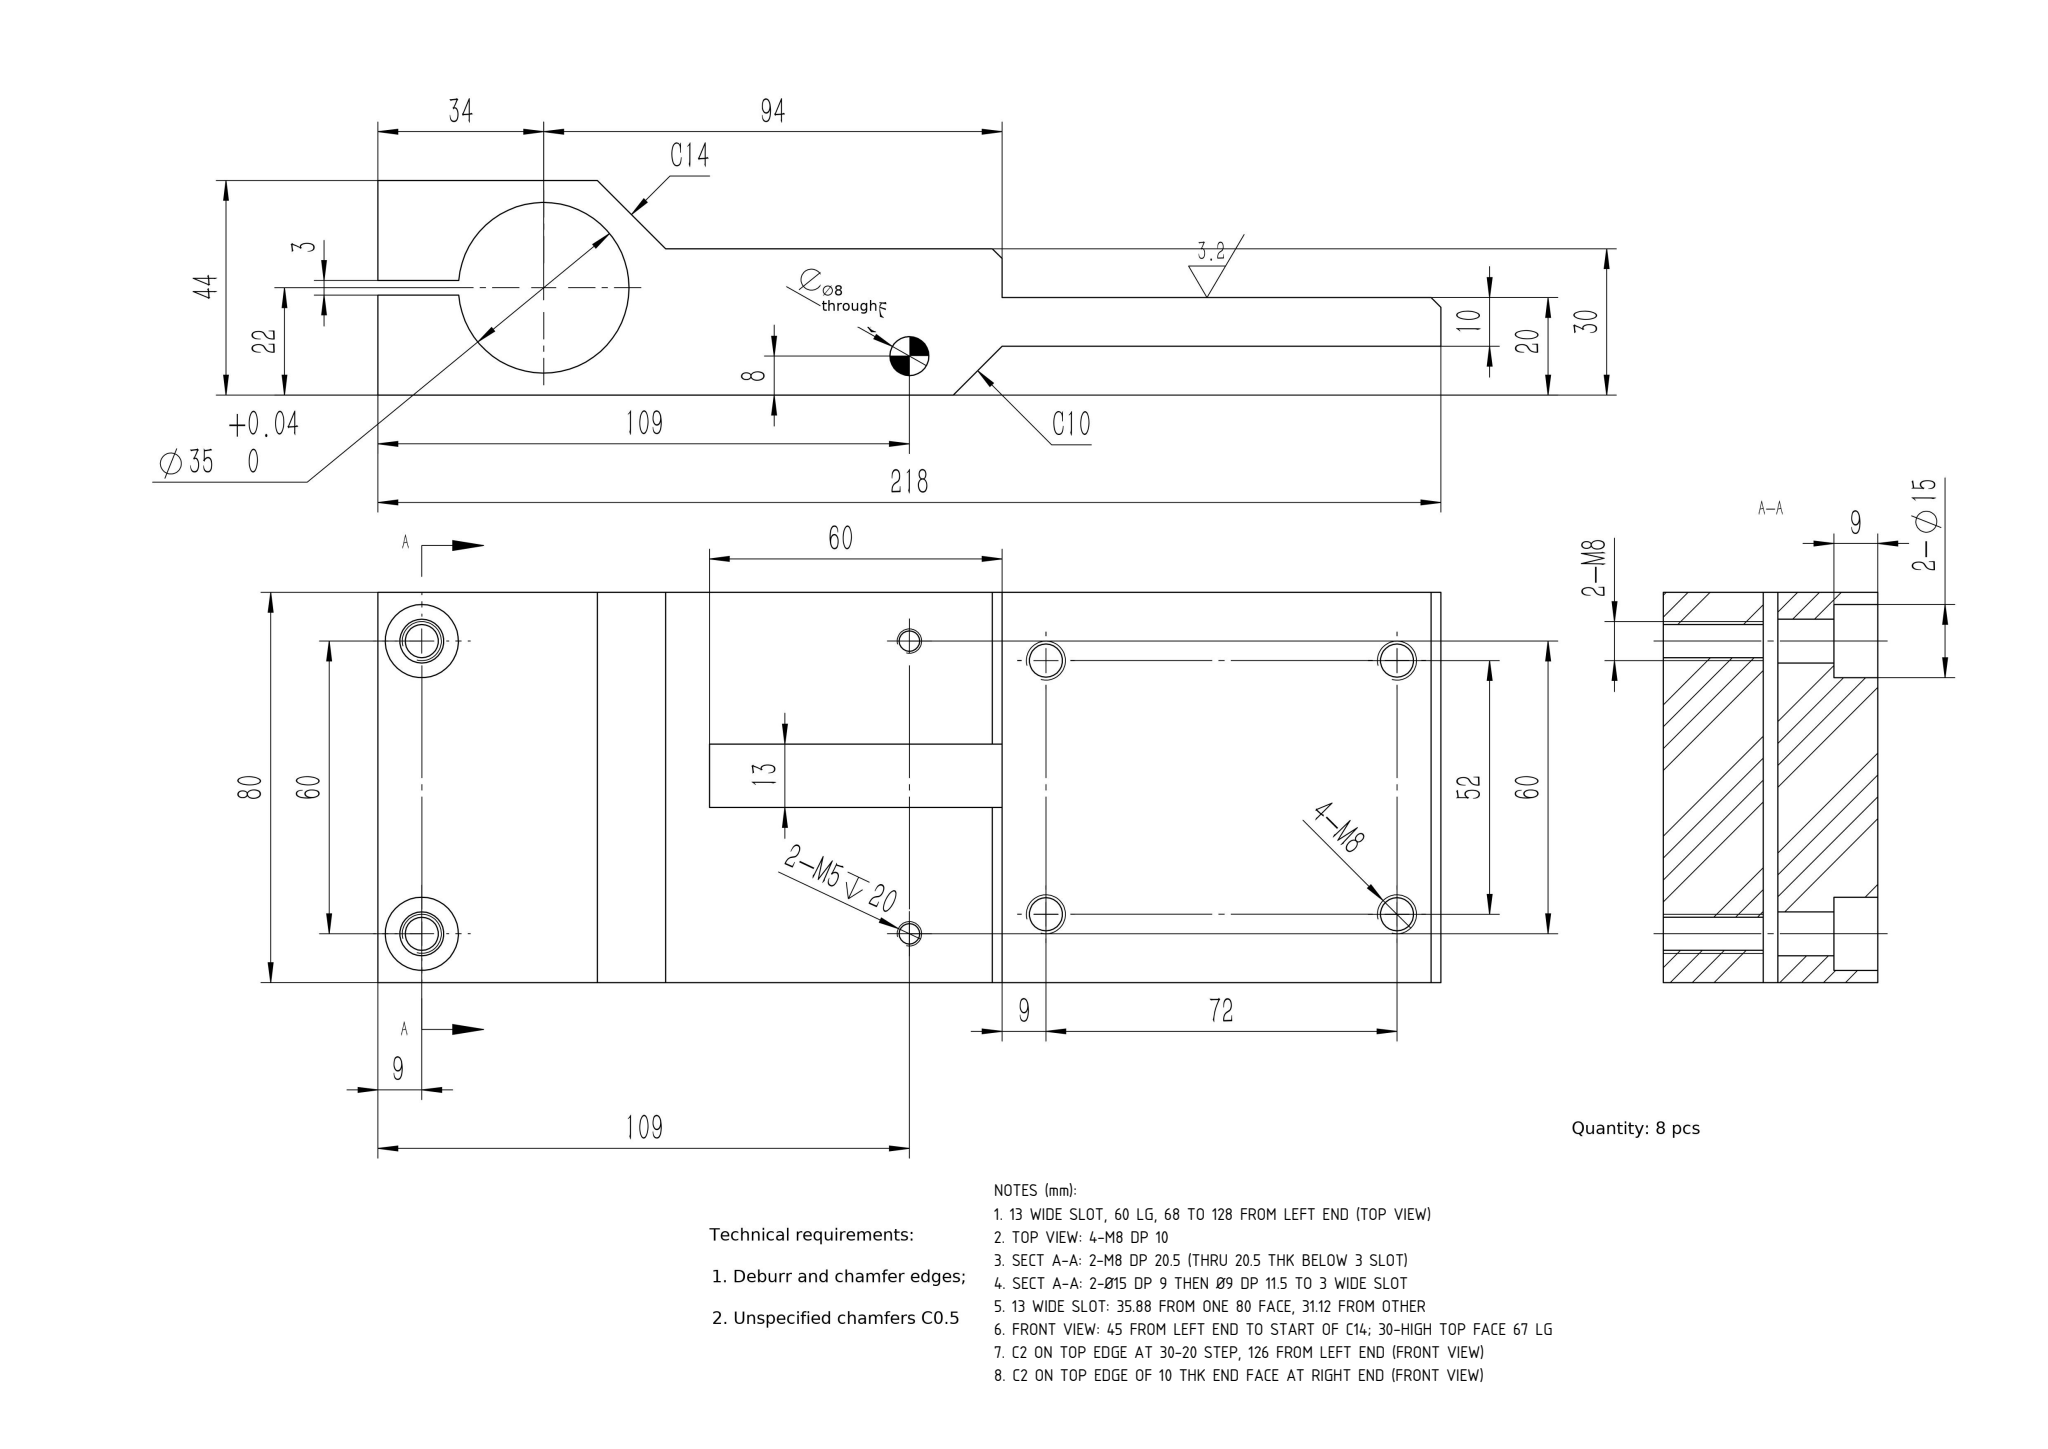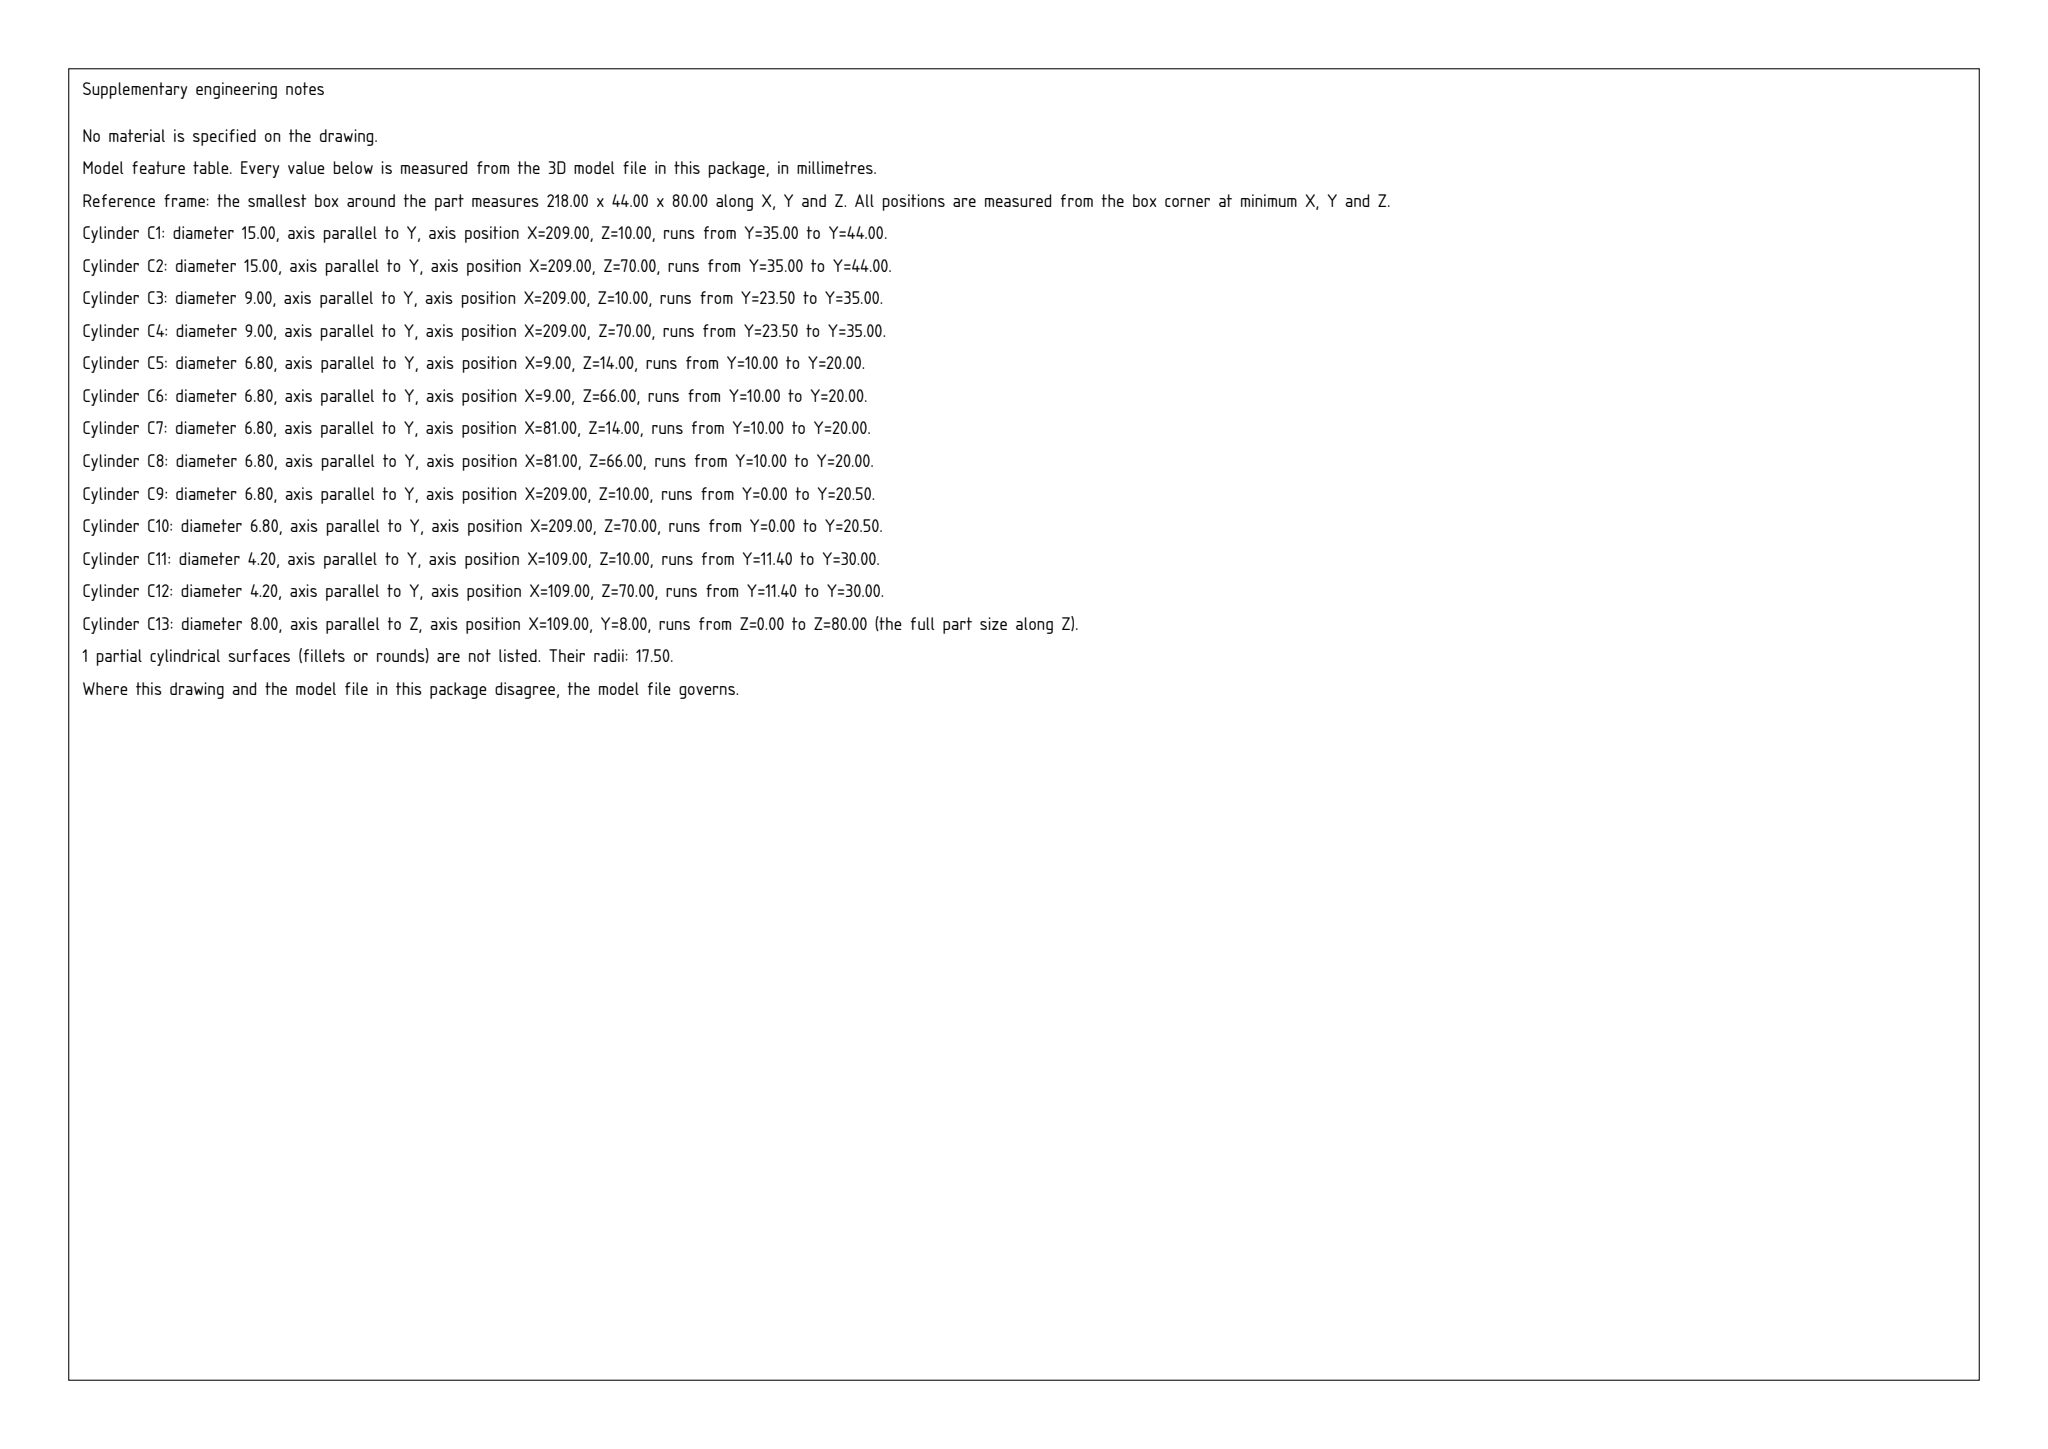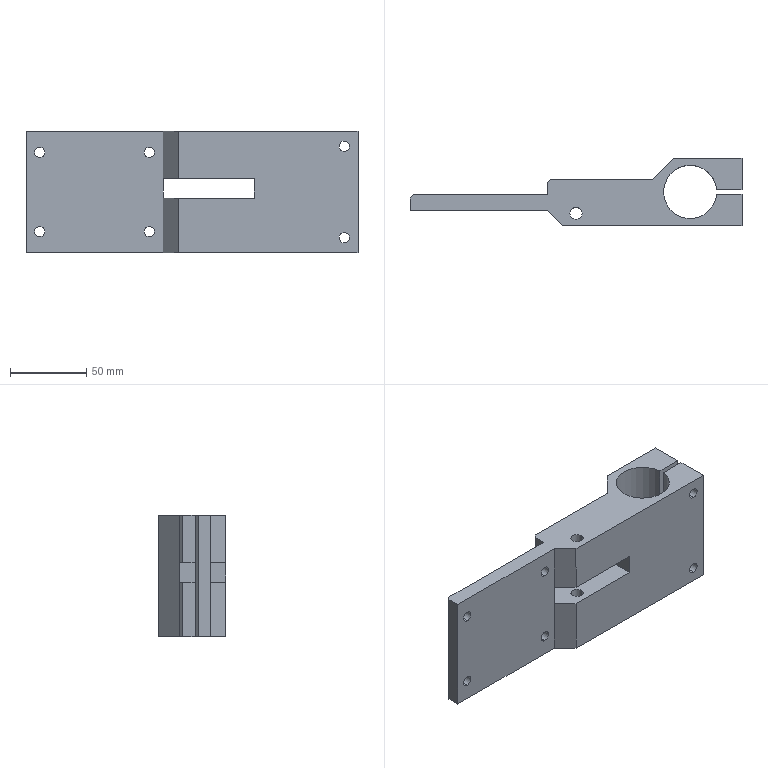Part | SolidWorks | mm | 1 solid | 56 faces | box 218 x 44 x 80 mm | volume 318006 mm3 | cylinder 30 | plane 26 | commonest cylinder face diameters 6.8 x12 4.2 x4 15 x4 9 x4 8 x4 35 x2
Drawing notes:
13 WIDE SLOT, 60 LG, 68 TO 128 FROM LEFT END (TOP VIEW) | from the solid: z-planes 35.88 & 48.88 = 13 apart; x-planes 90 & 150 = 60 apart, i.e. 68-128 from left end (218-150, 218-90); Ø8 THRU split 35.88+31.12
TOP VIEW: 4-M8 DP 10 | from the solid: Ø6.8 y-axis holes at x=9/81, z=14/66, length 10 (y30 to y20)
SECT A-A: 2-M8 DP 20.5 (THRU 20.5 THK BELOW 3 SLOT) | from the solid: Ø6.8 y-axis holes at x=209, z=10/70, length 20.5 (y20.5 to y0)
SECT A-A: 2-Ø15 DP 9 THEN Ø9 DP 11.5 TO 3 WIDE SLOT | from the solid: Ø15 L=9 (y44-35, planes y=35 x2) + Ø9 L=11.5 (y35-23.5) at x=209
13 WIDE SLOT: 35.88 FROM ONE 80 FACE, 31.12 FROM OTHER | from the solid: z planes 35.88 & 48.88; 80-48.88=31.12; Ø8 hole split L=35.88/31.12
FRONT VIEW: 45 FROM LEFT END TO START OF C14; 30-HIGH TOP FACE 67 LG | from the solid: Incl. plane 45° bbox_from [159,30,0] size 14x14x80; y=44 face x 173-218 (=45 from left end at x=218); y=30 face x 92-159 (=67 lg)
C2 ON TOP EDGE AT 30-20 STEP, 126 FROM LEFT END (FRONT VIEW) | from the solid: Incl. plane 45° bbox_from [90,28,0] size 2x2; 218-92=126 from left datum
C2 ON TOP EDGE OF 10 THK END FACE AT RIGHT END (FRONT VIEW) | from the solid: Incl. plane 45° bbox_from [0,18,0] size 2x2; end face x=0, y 10-18 (8 high)